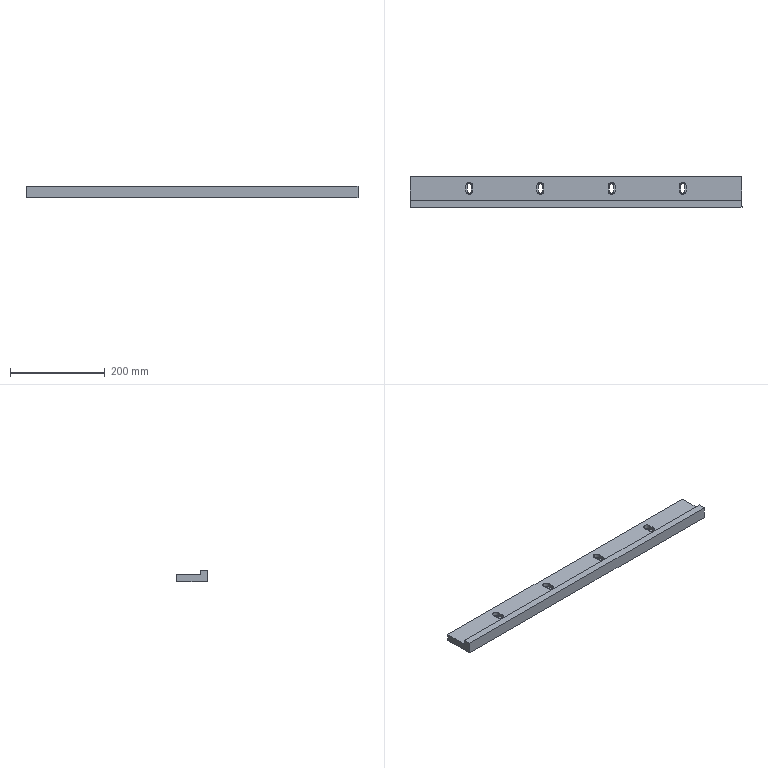Component | SolidWorks | LongSideFrameSupportB-1 | 1 solid | 52 faces | volume 771295 mm3 | plane 28 | cylinder 24 | commonest cylinder face diameters 15 x12 9 x12 | material Q235-A